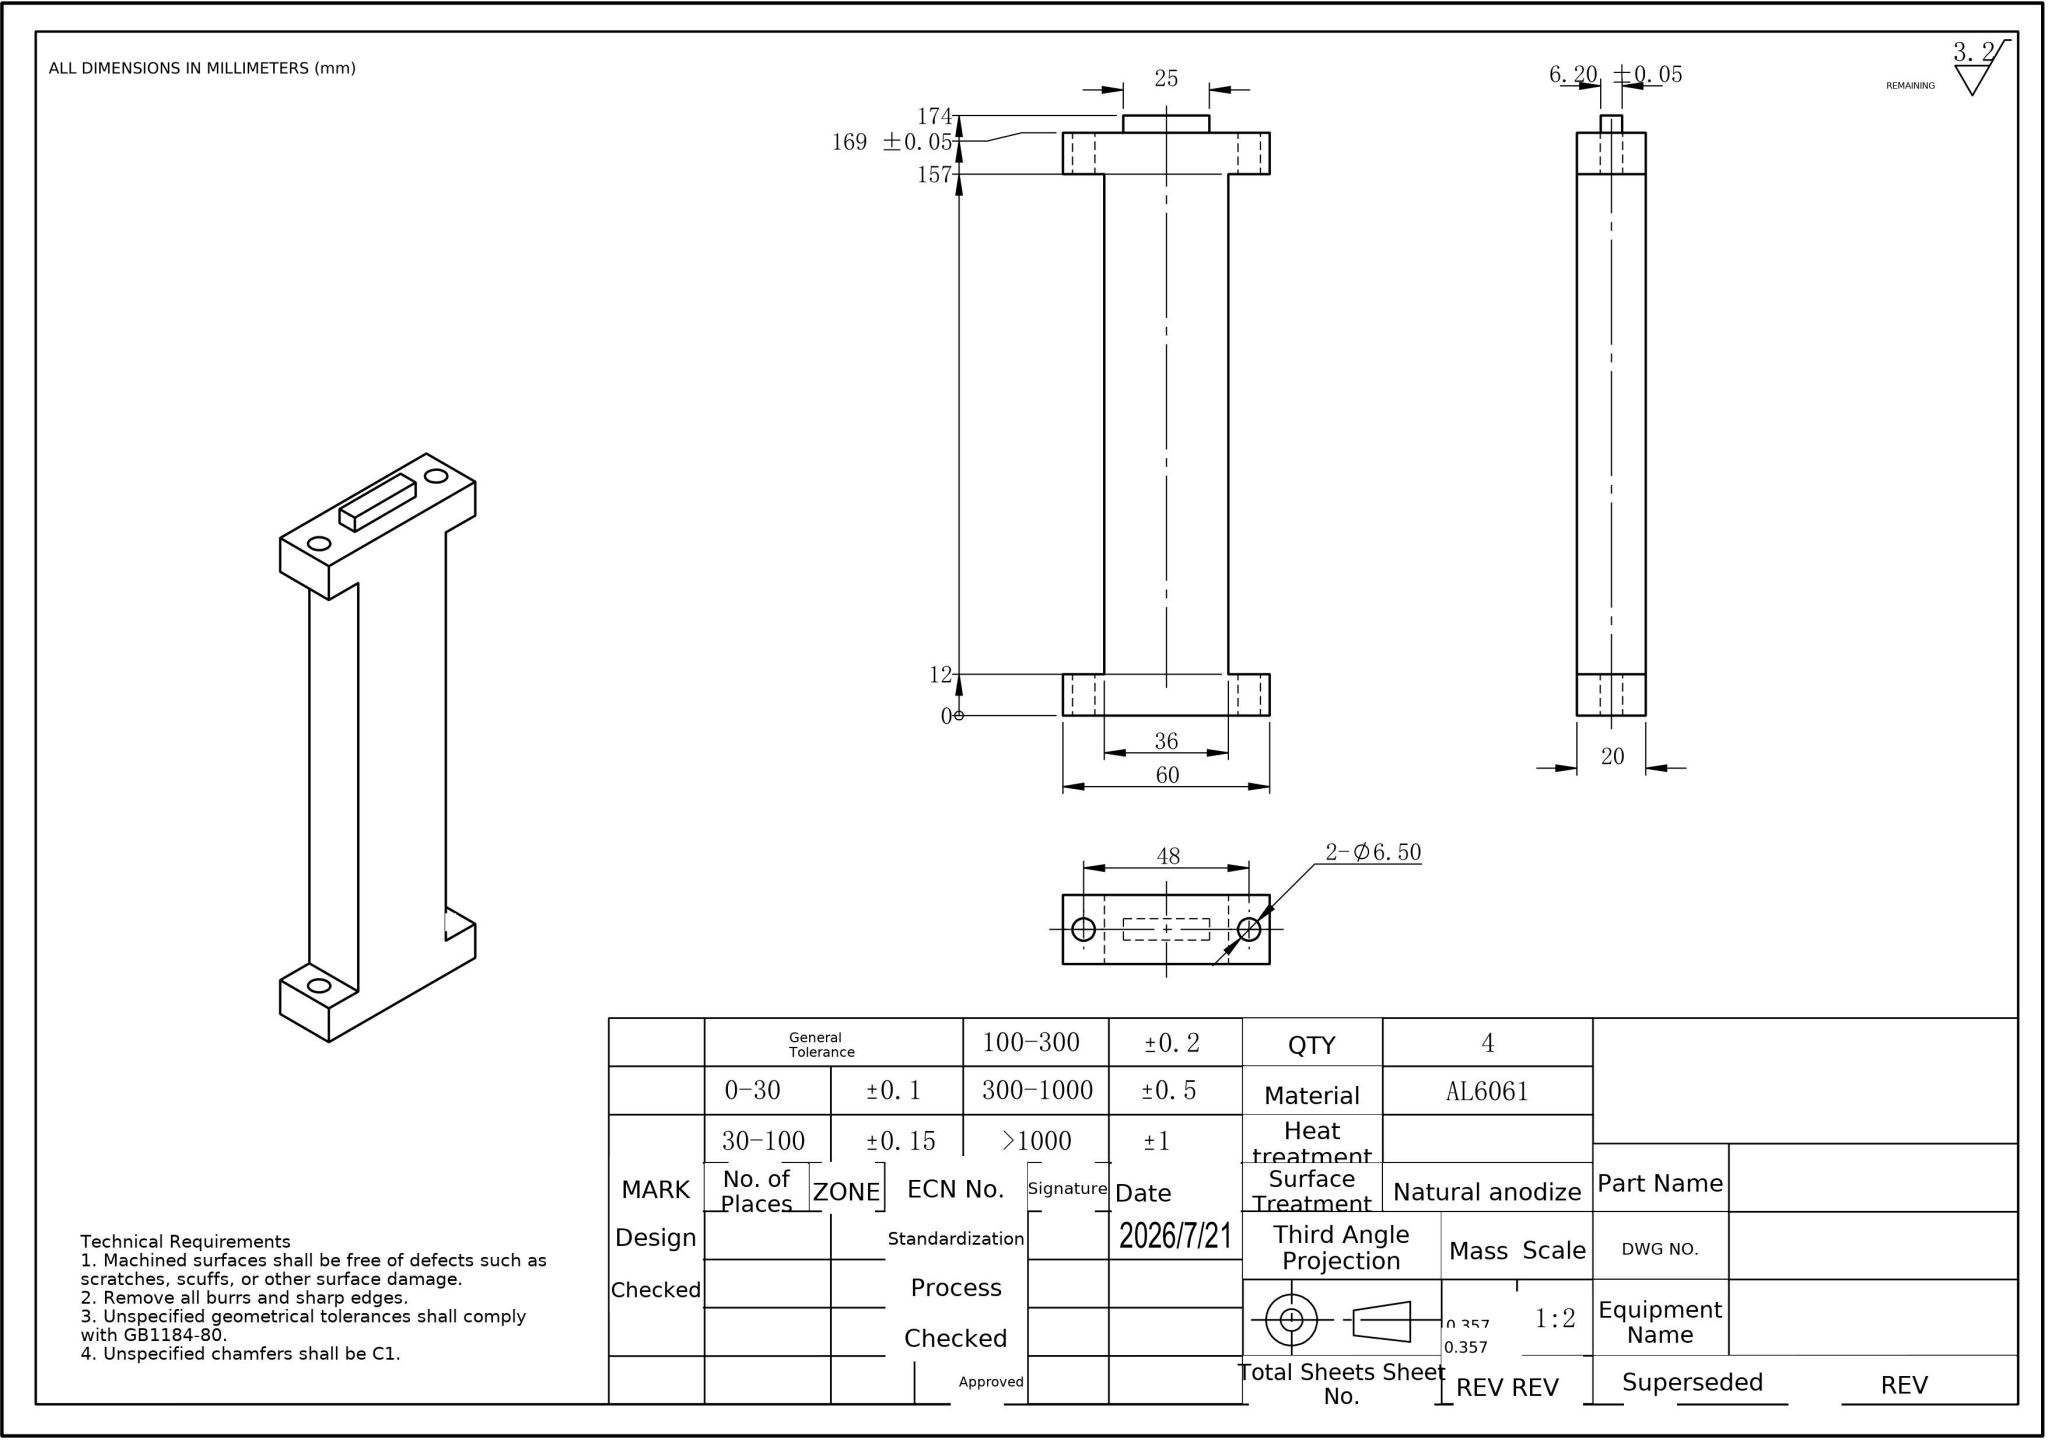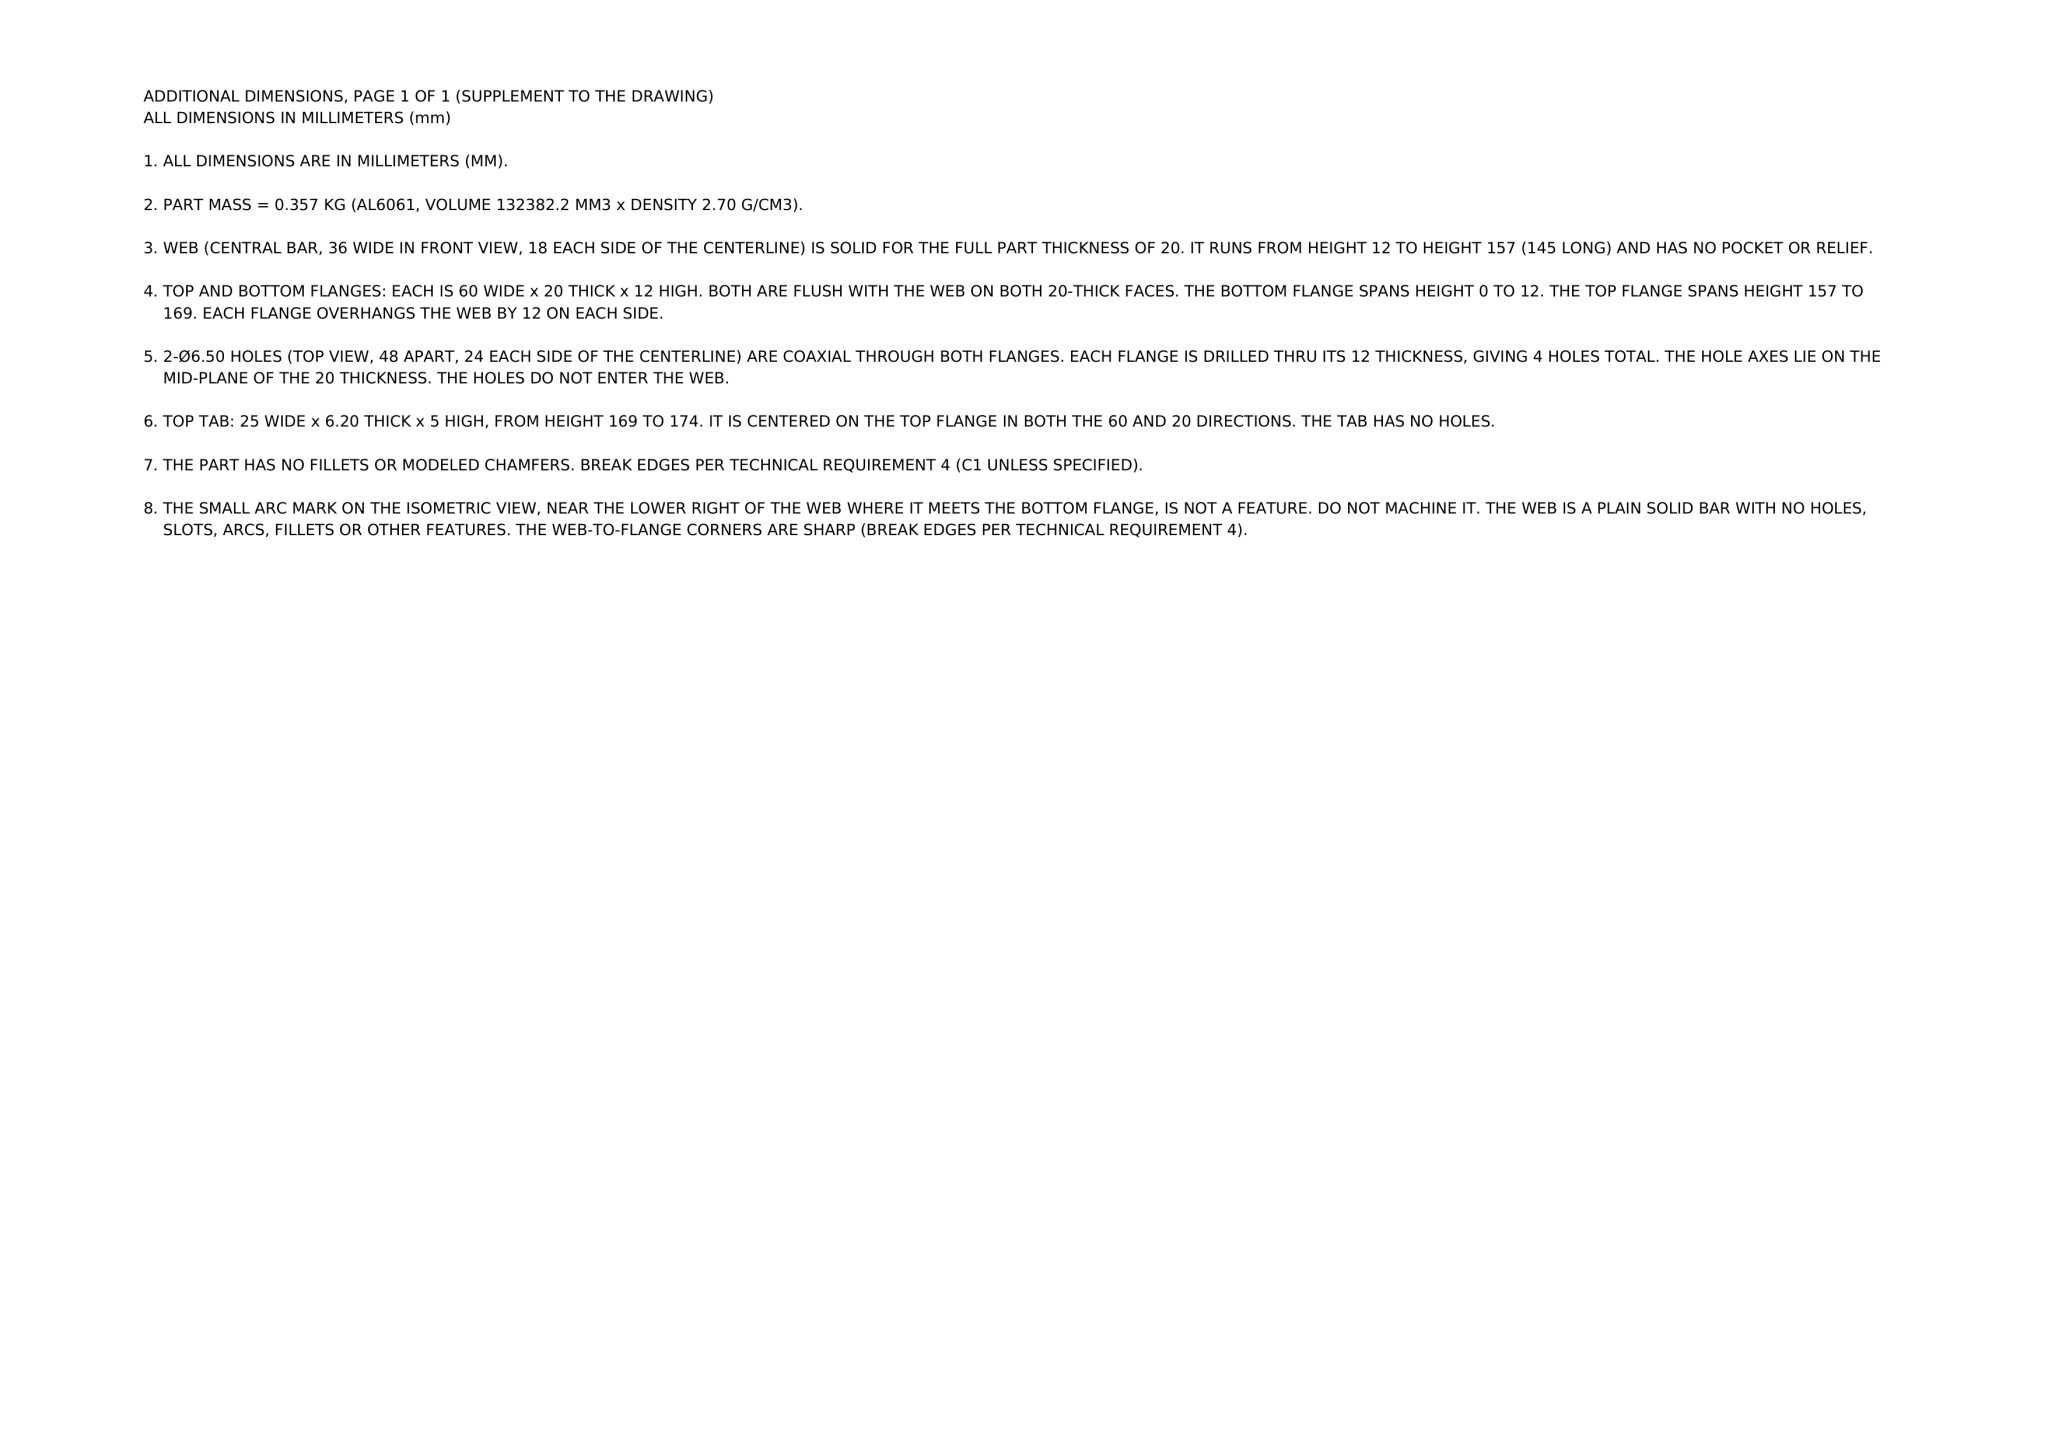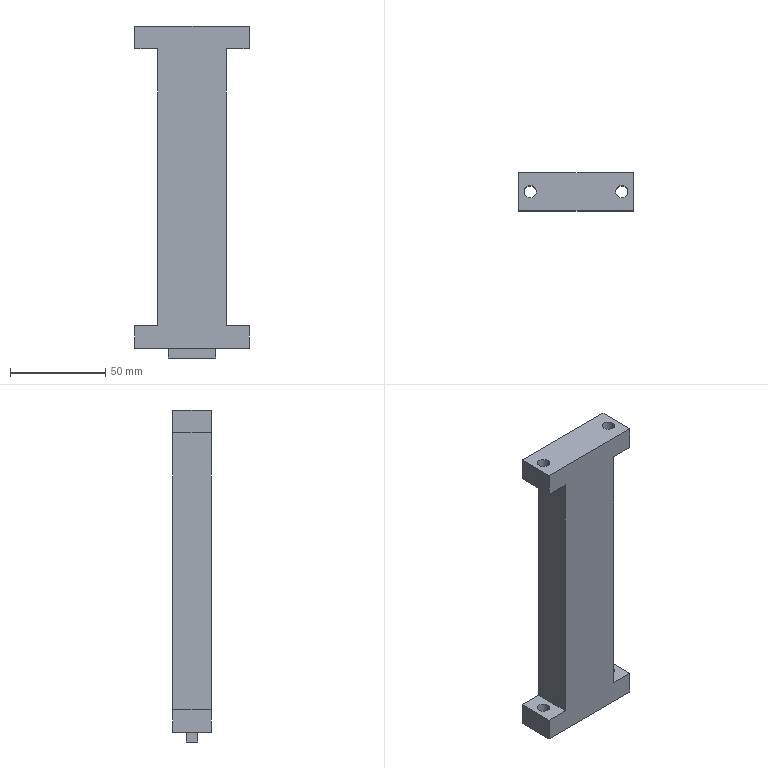Part | NX | mm | 1 solid | 27 faces | box 60 x 20 x 174 mm | volume 132382 mm3 | plane 19 | cylinder 8 | commonest cylinder face diameters 6.5 x8
STEP:
#1=COLOUR_RGB('',0.7922,0.8196,0.9333);
#2=FILL_AREA_STYLE_COLOUR('',#1);
#3=FILL_AREA_STYLE('',(#2));
#4=SURFACE_STYLE_FILL_AREA(#3);
#5=SURFACE_SIDE_STYLE('',(#4));
#6=SURFACE_STYLE_USAGE(.BOTH.,#5);
#7=PRESENTATION_STYLE_ASSIGNMENT((#6));
#8=CARTESIAN_POINT('',(27.25,-0.,-72.5));
#9=VERTEX_POINT('',#8);
#10=CARTESIAN_POINT('',(20.75,-0.,-72.5));
#11=VERTEX_POINT('',#10);
#12=CARTESIAN_POINT('',(24.,-0.,-72.5));
#13=DIRECTION('',(0.,0.,-1.));
#14=DIRECTION('',(-1.,0.,0.));
#15=AXIS2_PLACEMENT_3D('',#12,#13,#14);
#16=CIRCLE('',#15,3.25);
#17=EDGE_CURVE('',#9,#11,#16,.T.);
#18=ORIENTED_EDGE('',*,*,#17,.F.);
#19=CARTESIAN_POINT('',(27.25,-0.,-84.5));
#20=VERTEX_POINT('',#19);
#21=CARTESIAN_POINT('',(27.25,-0.,93.692));
#22=DIRECTION('',(0.,0.,-1.));
#23=VECTOR('',#22,1000.);
#24=LINE('',#21,#23);
#25=EDGE_CURVE('',#9,#20,#24,.T.);
#26=ORIENTED_EDGE('',*,*,#25,.T.);
#27=CARTESIAN_POINT('',(20.75,-0.,-84.5));
#28=VERTEX_POINT('',#27);
#29=CARTESIAN_POINT('',(24.,-0.,-84.5));
#30=DIRECTION('',(0.,0.,-1.));
#31=DIRECTION('',(1.,0.,0.));
#32=AXIS2_PLACEMENT_3D('',#29,#30,#31);
#33=CIRCLE('',#32,3.25);
#34=EDGE_CURVE('',#20,#28,#33,.T.);
#35=ORIENTED_EDGE('',*,*,#34,.T.);
#36=CARTESIAN_POINT('',(20.75,-0.,93.692));
#37=DIRECTION('',(0.,0.,-1.));
#38=VECTOR('',#37,1000.);
#39=LINE('',#36,#38);
#40=EDGE_CURVE('',#11,#28,#39,.T.);
#41=ORIENTED_EDGE('',*,*,#40,.F.);
#42=EDGE_LOOP('',(#18,#26,#35,#41));
#43=FACE_OUTER_BOUND('',#42,.T.);
#44=CARTESIAN_POINT('',(24.,-0.,93.692));
#45=DIRECTION('',(0.,0.,-1.));
#46=DIRECTION('',(-1.,0.,0.));
#47=AXIS2_PLACEMENT_3D('',#44,#45,#46);
#48=CYLINDRICAL_SURFACE('',#47,3.25);
#49=ADVANCED_FACE('',(#43),#48,.F.);
#50=CARTESIAN_POINT('',(20.75,-0.,84.5));
#51=VERTEX_POINT('',#50);
#52=CARTESIAN_POINT('',(27.25,-0.,84.5));
#53=VERTEX_POINT('',#52);
#54=CARTESIAN_POINT('',(24.,-0.,84.5));
#55=DIRECTION('',(0.,0.,1.));
#56=DIRECTION('',(-1.,0.,0.));
#57=AXIS2_PLACEMENT_3D('',#54,#55,#56);
#58=CIRCLE('',#57,3.25);
#59=EDGE_CURVE('',#51,#53,#58,.T.);
#60=ORIENTED_EDGE('',*,*,#59,.T.);
#61=CARTESIAN_POINT('',(27.25,-0.,72.5));
#62=VERTEX_POINT('',#61);
#63=CARTESIAN_POINT('',(27.25,-0.,93.692));
#64=DIRECTION('',(0.,0.,-1.));
#65=VECTOR('',#64,1000.);
#66=LINE('',#63,#65);
#67=EDGE_CURVE('',#53,#62,#66,.T.);
#68=ORIENTED_EDGE('',*,*,#67,.T.);
#69=CARTESIAN_POINT('',(20.75,-0.,72.5));
#70=VERTEX_POINT('',#69);
#71=CARTESIAN_POINT('',(24.,-0.,72.5));
#72=DIRECTION('',(-0.,0.,1.));
#73=DIRECTION('',(1.,0.,0.));
#74=AXIS2_PLACEMENT_3D('',#71,#72,#73);
#75=CIRCLE('',#74,3.25);
#76=EDGE_CURVE('',#70,#62,#75,.T.);
#77=ORIENTED_EDGE('',*,*,#76,.F.);
#78=CARTESIAN_POINT('',(20.75,-0.,93.692));
#79=DIRECTION('',(0.,0.,-1.));
#80=VECTOR('',#79,1000.);
#81=LINE('',#78,#80);
#82=EDGE_CURVE('',#51,#70,#81,.T.);
#83=ORIENTED_EDGE('',*,*,#82,.F.);
#84=EDGE_LOOP('',(#60,#68,#77,#83));
#85=FACE_OUTER_BOUND('',#84,.T.);
#86=CARTESIAN_POINT('',(24.,-0.,93.692));
#87=DIRECTION('',(0.,0.,-1.));
#88=DIRECTION('',(-1.,0.,0.));
#89=AXIS2_PLACEMENT_3D('',#86,#87,#88);
#90=CYLINDRICAL_SURFACE('',#89,3.25);
#91=ADVANCED_FACE('',(#85),#90,.F.);
#92=CARTESIAN_POINT('',(-27.25,-0.,84.5));
#93=VERTEX_POINT('',#92);
#94=CARTESIAN_POINT('',(-20.75,0.,84.5));
#95=VERTEX_POINT('',#94);
#96=CARTESIAN_POINT('',(-24.,-0.,84.5));
#97=DIRECTION('',(0.,0.,1.));
#98=DIRECTION('',(-1.,0.,0.));
#99=AXIS2_PLACEMENT_3D('',#96,#97,#98);
#100=CIRCLE('',#99,3.25);
#101=EDGE_CURVE('',#93,#95,#100,.T.);
#102=ORIENTED_EDGE('',*,*,#101,.T.);
#103=CARTESIAN_POINT('',(-20.75,0.,72.5));
#104=VERTEX_POINT('',#103);
#105=CARTESIAN_POINT('',(-20.75,0.,93.692));
#106=DIRECTION('',(0.,0.,-1.));
#107=VECTOR('',#106,1000.);
#108=LINE('',#105,#107);
#109=EDGE_CURVE('',#95,#104,#108,.T.);
#110=ORIENTED_EDGE('',*,*,#109,.T.);
#111=CARTESIAN_POINT('',(-27.25,-0.,72.5));
#112=VERTEX_POINT('',#111);
#113=CARTESIAN_POINT('',(-24.,-0.,72.5));
#114=DIRECTION('',(0.,0.,1.));
#115=DIRECTION('',(1.,0.,0.));
#116=AXIS2_PLACEMENT_3D('',#113,#114,#115);
#117=CIRCLE('',#116,3.25);
#118=EDGE_CURVE('',#112,#104,#117,.T.);
#119=ORIENTED_EDGE('',*,*,#118,.F.);
#120=CARTESIAN_POINT('',(-27.25,-0.,93.692));
#121=DIRECTION('',(0.,0.,-1.));
#122=VECTOR('',#121,1000.);
#123=LINE('',#120,#122);
#124=EDGE_CURVE('',#93,#112,#123,.T.);
#125=ORIENTED_EDGE('',*,*,#124,.F.);
#126=EDGE_LOOP('',(#102,#110,#119,#125));
#127=FACE_OUTER_BOUND('',#126,.T.);
#128=CARTESIAN_POINT('',(-24.,-0.,93.692));
#129=DIRECTION('',(0.,0.,-1.));
#130=DIRECTION('',(-1.,0.,0.));
#131=AXIS2_PLACEMENT_3D('',#128,#129,#130);
#132=CYLINDRICAL_SURFACE('',#131,3.25);
#133=ADVANCED_FACE('',(#127),#132,.F.);
#134=CARTESIAN_POINT('',(-20.75,0.,-72.5));
#135=VERTEX_POINT('',#134);
#136=CARTESIAN_POINT('',(-27.25,-0.,-72.5));
#137=VERTEX_POINT('',#136);
#138=CARTESIAN_POINT('',(-24.,-0.,-72.5));
#139=DIRECTION('',(0.,0.,-1.));
#140=DIRECTION('',(-1.,0.,0.));
#141=AXIS2_PLACEMENT_3D('',#138,#139,#140);
#142=CIRCLE('',#141,3.25);
#143=EDGE_CURVE('',#135,#137,#142,.T.);
#144=ORIENTED_EDGE('',*,*,#143,.F.);
#145=CARTESIAN_POINT('',(-20.75,0.,-84.5));
#146=VERTEX_POINT('',#145);
#147=CARTESIAN_POINT('',(-20.75,0.,93.692));
#148=DIRECTION('',(0.,0.,-1.));
#149=VECTOR('',#148,1000.);
#150=LINE('',#147,#149);
#151=EDGE_CURVE('',#135,#146,#150,.T.);
#152=ORIENTED_EDGE('',*,*,#151,.T.);
#153=CARTESIAN_POINT('',(-27.25,-0.,-84.5));
#154=VERTEX_POINT('',#153);
#155=CARTESIAN_POINT('',(-24.,-0.,-84.5));
#156=DIRECTION('',(0.,0.,-1.));
#157=DIRECTION('',(-1.,0.,0.));
#158=AXIS2_PLACEMENT_3D('',#155,#156,#157);
#159=CIRCLE('',#158,3.25);
#160=EDGE_CURVE('',#146,#154,#159,.T.);
#161=ORIENTED_EDGE('',*,*,#160,.T.);
#162=CARTESIAN_POINT('',(-27.25,-0.,93.692));
#163=DIRECTION('',(0.,0.,-1.));
#164=VECTOR('',#163,1000.);
#165=LINE('',#162,#164);
#166=EDGE_CURVE('',#137,#154,#165,.T.);
#167=ORIENTED_EDGE('',*,*,#166,.F.);
#168=EDGE_LOOP('',(#144,#152,#161,#167));
#169=FACE_OUTER_BOUND('',#168,.T.);
#170=CARTESIAN_POINT('',(-24.,-0.,93.692));
#171=DIRECTION('',(0.,0.,-1.));
#172=DIRECTION('',(-1.,0.,0.));
#173=AXIS2_PLACEMENT_3D('',#170,#171,#172);
#174=CYLINDRICAL_SURFACE('',#173,3.25);
#175=ADVANCED_FACE('',(#169),#174,.F.);
#176=CARTESIAN_POINT('',(24.,-0.,-84.5));
#177=DIRECTION('',(0.,0.,-1.));
#178=DIRECTION('',(1.,0.,0.));
#179=AXIS2_PLACEMENT_3D('',#176,#177,#178);
#180=CIRCLE('',#179,3.25);
#181=EDGE_CURVE('',#28,#20,#180,.T.);
#182=ORIENTED_EDGE('',*,*,#181,.F.);
#183=ORIENTED_EDGE('',*,*,#34,.F.);
#184=EDGE_LOOP('',(#182,#183));
#185=FACE_BOUND('',#184,.T.);
#186=CARTESIAN_POINT('',(-24.,-0.,-84.5));
#187=DIRECTION('',(0.,0.,-1.));
#188=DIRECTION('',(-1.,0.,0.));
#189=AXIS2_PLACEMENT_3D('',#186,#187,#188);
#190=CIRCLE('',#189,3.25);
#191=EDGE_CURVE('',#154,#146,#190,.T.);
#192=ORIENTED_EDGE('',*,*,#191,.F.);
#193=ORIENTED_EDGE('',*,*,#160,.F.);
#194=EDGE_LOOP('',(#192,#193));
#195=FACE_BOUND('',#194,.T.);
#196=CARTESIAN_POINT('',(30.,-10.,-84.5));
#197=VERTEX_POINT('',#196);
#198=CARTESIAN_POINT('',(-30.,-10.,-84.5));
#199=VERTEX_POINT('',#198);
#200=CARTESIAN_POINT('',(-30.,-10.,-84.5));
#201=DIRECTION('',(-1.,0.,0.));
#202=VECTOR('',#201,1000.);
#203=LINE('',#200,#202);
#204=EDGE_CURVE('',#197,#199,#203,.T.);
#205=ORIENTED_EDGE('',*,*,#204,.T.);
#206=CARTESIAN_POINT('',(-30.,10.,-84.5));
#207=VERTEX_POINT('',#206);
#208=CARTESIAN_POINT('',(-30.,10.,-84.5));
#209=DIRECTION('',(0.,-1.,0.));
#210=VECTOR('',#209,1000.);
#211=LINE('',#208,#210);
#212=EDGE_CURVE('',#207,#199,#211,.T.);
#213=ORIENTED_EDGE('',*,*,#212,.F.);
#214=CARTESIAN_POINT('',(30.,10.,-84.5));
#215=VERTEX_POINT('',#214);
#216=CARTESIAN_POINT('',(-30.,10.,-84.5));
#217=DIRECTION('',(-1.,0.,0.));
#218=VECTOR('',#217,1000.);
#219=LINE('',#216,#218);
#220=EDGE_CURVE('',#215,#207,#219,.T.);
#221=ORIENTED_EDGE('',*,*,#220,.F.);
#222=CARTESIAN_POINT('',(30.,10.,-84.5));
#223=DIRECTION('',(0.,-1.,0.));
#224=VECTOR('',#223,1000.);
#225=LINE('',#222,#224);
#226=EDGE_CURVE('',#215,#197,#225,.T.);
#227=ORIENTED_EDGE('',*,*,#226,.T.);
#228=EDGE_LOOP('',(#205,#213,#221,#227));
#229=FACE_OUTER_BOUND('',#228,.T.);
#230=CARTESIAN_POINT('',(-12.5,-3.1,-84.5));
#231=VERTEX_POINT('',#230);
#232=CARTESIAN_POINT('',(-12.5,3.1,-84.5));
#233=VERTEX_POINT('',#232);
#234=CARTESIAN_POINT('',(-12.5,-3.1,-84.5));
#235=DIRECTION('',(0.,1.,0.));
#236=VECTOR('',#235,1000.);
#237=LINE('',#234,#236);
#238=EDGE_CURVE('',#231,#233,#237,.T.);
#239=ORIENTED_EDGE('',*,*,#238,.F.);
#240=CARTESIAN_POINT('',(12.5,-3.1,-84.5));
#241=VERTEX_POINT('',#240);
#242=CARTESIAN_POINT('',(12.5,-3.1,-84.5));
#243=DIRECTION('',(-1.,0.,0.));
#244=VECTOR('',#243,1000.);
#245=LINE('',#242,#244);
#246=EDGE_CURVE('',#241,#231,#245,.T.);
#247=ORIENTED_EDGE('',*,*,#246,.F.);
#248=CARTESIAN_POINT('',(12.5,3.1,-84.5));
#249=VERTEX_POINT('',#248);
#250=CARTESIAN_POINT('',(12.5,-3.1,-84.5));
#251=DIRECTION('',(0.,-1.,0.));
#252=VECTOR('',#251,1000.);
#253=LINE('',#250,#252);
#254=EDGE_CURVE('',#249,#241,#253,.T.);
#255=ORIENTED_EDGE('',*,*,#254,.F.);
#256=CARTESIAN_POINT('',(12.5,3.1,-84.5));
#257=DIRECTION('',(1.,0.,0.));
#258=VECTOR('',#257,1000.);
#259=LINE('',#256,#258);
#260=EDGE_CURVE('',#233,#249,#259,.T.);
#261=ORIENTED_EDGE('',*,*,#260,.F.);
#262=EDGE_LOOP('',(#239,#247,#255,#261));
#263=FACE_BOUND('',#262,.T.);
#264=CARTESIAN_POINT('',(-30.,10.,-84.5));
#265=DIRECTION('',(0.,0.,1.));
#266=DIRECTION('',(1.,0.,0.));
#267=AXIS2_PLACEMENT_3D('',#264,#265,#266);
#268=PLANE('',#267);
#269=ADVANCED_FACE('',(#185,#195,#229,#263),#268,.F.);
#270=CARTESIAN_POINT('',(30.,10.,-72.5));
#271=VERTEX_POINT('',#270);
#272=CARTESIAN_POINT('',(30.,10.,84.5));
#273=DIRECTION('',(0.,0.,-1.));
#274=VECTOR('',#273,1000.);
#275=LINE('',#272,#274);
#276=EDGE_CURVE('',#271,#215,#275,.T.);
#277=ORIENTED_EDGE('',*,*,#276,.F.);
#278=CARTESIAN_POINT('',(30.,-10.,-72.5));
#279=VERTEX_POINT('',#278);
#280=CARTESIAN_POINT('',(30.,10.,-72.5));
#281=DIRECTION('',(0.,-1.,0.));
#282=VECTOR('',#281,1000.);
#283=LINE('',#280,#282);
#284=EDGE_CURVE('',#271,#279,#283,.T.);
#285=ORIENTED_EDGE('',*,*,#284,.T.);
#286=CARTESIAN_POINT('',(30.,-10.,84.5));
#287=DIRECTION('',(0.,0.,-1.));
#288=VECTOR('',#287,1000.);
#289=LINE('',#286,#288);
#290=EDGE_CURVE('',#279,#197,#289,.T.);
#291=ORIENTED_EDGE('',*,*,#290,.T.);
#292=ORIENTED_EDGE('',*,*,#226,.F.);
#293=EDGE_LOOP('',(#277,#285,#291,#292));
#294=FACE_OUTER_BOUND('',#293,.T.);
#295=CARTESIAN_POINT('',(30.,10.,84.5));
#296=DIRECTION('',(-1.,0.,0.));
#297=DIRECTION('',(0.,0.,1.));
#298=AXIS2_PLACEMENT_3D('',#295,#296,#297);
#299=PLANE('',#298);
#300=ADVANCED_FACE('',(#294),#299,.F.);
#301=CARTESIAN_POINT('',(-30.,10.,72.5));
#302=VERTEX_POINT('',#301);
#303=CARTESIAN_POINT('',(-30.,10.,84.5));
#304=VERTEX_POINT('',#303);
#305=CARTESIAN_POINT('',(-30.,10.,84.5));
#306=DIRECTION('',(0.,0.,1.));
#307=VECTOR('',#306,1000.);
#308=LINE('',#305,#307);
#309=EDGE_CURVE('',#302,#304,#308,.T.);
#310=ORIENTED_EDGE('',*,*,#309,.F.);
#311=CARTESIAN_POINT('',(-30.,-10.,72.5));
#312=VERTEX_POINT('',#311);
#313=CARTESIAN_POINT('',(-30.,10.,72.5));
#314=DIRECTION('',(0.,-1.,0.));
#315=VECTOR('',#314,1000.);
#316=LINE('',#313,#315);
#317=EDGE_CURVE('',#302,#312,#316,.T.);
#318=ORIENTED_EDGE('',*,*,#317,.T.);
#319=CARTESIAN_POINT('',(-30.,-10.,84.5));
#320=VERTEX_POINT('',#319);
#321=CARTESIAN_POINT('',(-30.,-10.,84.5));
#322=DIRECTION('',(0.,0.,1.));
#323=VECTOR('',#322,1000.);
#324=LINE('',#321,#323);
#325=EDGE_CURVE('',#312,#320,#324,.T.);
#326=ORIENTED_EDGE('',*,*,#325,.T.);
#327=CARTESIAN_POINT('',(-30.,10.,84.5));
#328=DIRECTION('',(0.,-1.,0.));
#329=VECTOR('',#328,1000.);
#330=LINE('',#327,#329);
#331=EDGE_CURVE('',#304,#320,#330,.T.);
#332=ORIENTED_EDGE('',*,*,#331,.F.);
#333=EDGE_LOOP('',(#310,#318,#326,#332));
#334=FACE_OUTER_BOUND('',#333,.T.);
#335=CARTESIAN_POINT('',(-30.,10.,84.5));
#336=DIRECTION('',(1.,0.,0.));
#337=DIRECTION('',(0.,0.,-1.));
#338=AXIS2_PLACEMENT_3D('',#335,#336,#337);
#339=PLANE('',#338);
#340=ADVANCED_FACE('',(#334),#339,.F.);
#341=CARTESIAN_POINT('',(30.,-10.,84.5));
#342=VERTEX_POINT('',#341);
#343=CARTESIAN_POINT('',(30.,-10.,72.5));
#344=VERTEX_POINT('',#343);
#345=CARTESIAN_POINT('',(30.,-10.,84.5));
#346=DIRECTION('',(0.,0.,-1.));
#347=VECTOR('',#346,1000.);
#348=LINE('',#345,#347);
#349=EDGE_CURVE('',#342,#344,#348,.T.);
#350=ORIENTED_EDGE('',*,*,#349,.T.);
#351=CARTESIAN_POINT('',(30.,10.,72.5));
#352=VERTEX_POINT('',#351);
#353=CARTESIAN_POINT('',(30.,10.,72.5));
#354=DIRECTION('',(0.,-1.,0.));
#355=VECTOR('',#354,1000.);
#356=LINE('',#353,#355);
#357=EDGE_CURVE('',#352,#344,#356,.T.);
#358=ORIENTED_EDGE('',*,*,#357,.F.);
#359=CARTESIAN_POINT('',(30.,10.,84.5));
#360=VERTEX_POINT('',#359);
#361=CARTESIAN_POINT('',(30.,10.,84.5));
#362=DIRECTION('',(0.,0.,-1.));
#363=VECTOR('',#362,1000.);
#364=LINE('',#361,#363);
#365=EDGE_CURVE('',#360,#352,#364,.T.);
#366=ORIENTED_EDGE('',*,*,#365,.F.);
#367=CARTESIAN_POINT('',(30.,10.,84.5));
#368=DIRECTION('',(0.,-1.,0.));
#369=VECTOR('',#368,1000.);
#370=LINE('',#367,#369);
#371=EDGE_CURVE('',#360,#342,#370,.T.);
#372=ORIENTED_EDGE('',*,*,#371,.T.);
#373=EDGE_LOOP('',(#350,#358,#366,#372));
#374=FACE_OUTER_BOUND('',#373,.T.);
#375=CARTESIAN_POINT('',(30.,10.,84.5));
#376=DIRECTION('',(-1.,0.,0.));
#377=DIRECTION('',(0.,0.,1.));
#378=AXIS2_PLACEMENT_3D('',#375,#376,#377);
#379=PLANE('',#378);
#380=ADVANCED_FACE('',(#374),#379,.F.);
#381=CARTESIAN_POINT('',(-30.,-10.,-72.5));
#382=VERTEX_POINT('',#381);
#383=CARTESIAN_POINT('',(-30.,-10.,84.5));
#384=DIRECTION('',(0.,0.,1.));
#385=VECTOR('',#384,1000.);
#386=LINE('',#383,#385);
#387=EDGE_CURVE('',#199,#382,#386,.T.);
#388=ORIENTED_EDGE('',*,*,#387,.T.);
#389=CARTESIAN_POINT('',(-30.,10.,-72.5));
#390=VERTEX_POINT('',#389);
#391=CARTESIAN_POINT('',(-30.,10.,-72.5));
#392=DIRECTION('',(0.,-1.,0.));
#393=VECTOR('',#392,1000.);
#394=LINE('',#391,#393);
#395=EDGE_CURVE('',#390,#382,#394,.T.);
#396=ORIENTED_EDGE('',*,*,#395,.F.);
#397=CARTESIAN_POINT('',(-30.,10.,84.5));
#398=DIRECTION('',(0.,0.,1.));
#399=VECTOR('',#398,1000.);
#400=LINE('',#397,#399);
#401=EDGE_CURVE('',#207,#390,#400,.T.);
#402=ORIENTED_EDGE('',*,*,#401,.F.);
#403=ORIENTED_EDGE('',*,*,#212,.T.);
#404=EDGE_LOOP('',(#388,#396,#402,#403));
#405=FACE_OUTER_BOUND('',#404,.T.);
#406=CARTESIAN_POINT('',(-30.,10.,84.5));
#407=DIRECTION('',(1.,0.,0.));
#408=DIRECTION('',(0.,0.,-1.));
#409=AXIS2_PLACEMENT_3D('',#406,#407,#408);
#410=PLANE('',#409);
#411=ADVANCED_FACE('',(#405),#410,.F.);
#412=ORIENTED_EDGE('',*,*,#59,.F.);
#413=CARTESIAN_POINT('',(24.,-0.,84.5));
#414=DIRECTION('',(0.,0.,1.));
#415=DIRECTION('',(-1.,0.,0.));
#416=AXIS2_PLACEMENT_3D('',#413,#414,#415);
#417=CIRCLE('',#416,3.25);
#418=EDGE_CURVE('',#53,#51,#417,.T.);
#419=ORIENTED_EDGE('',*,*,#418,.F.);
#420=EDGE_LOOP('',(#412,#419));
#421=FACE_BOUND('',#420,.T.);
#422=ORIENTED_EDGE('',*,*,#101,.F.);
#423=CARTESIAN_POINT('',(-24.,-0.,84.5));
#424=DIRECTION('',(0.,0.,1.));
#425=DIRECTION('',(-1.,0.,0.));
#426=AXIS2_PLACEMENT_3D('',#423,#424,#425);
#427=CIRCLE('',#426,3.25);
#428=EDGE_CURVE('',#95,#93,#427,.T.);
#429=ORIENTED_EDGE('',*,*,#428,.F.);
#430=EDGE_LOOP('',(#422,#429));
#431=FACE_BOUND('',#430,.T.);
#432=CARTESIAN_POINT('',(-30.,-10.,84.5));
#433=DIRECTION('',(1.,0.,0.));
#434=VECTOR('',#433,1000.);
#435=LINE('',#432,#434);
#436=EDGE_CURVE('',#320,#342,#435,.T.);
#437=ORIENTED_EDGE('',*,*,#436,.T.);
#438=ORIENTED_EDGE('',*,*,#371,.F.);
#439=CARTESIAN_POINT('',(-30.,10.,84.5));
#440=DIRECTION('',(1.,0.,0.));
#441=VECTOR('',#440,1000.);
#442=LINE('',#439,#441);
#443=EDGE_CURVE('',#304,#360,#442,.T.);
#444=ORIENTED_EDGE('',*,*,#443,.F.);
#445=ORIENTED_EDGE('',*,*,#331,.T.);
#446=EDGE_LOOP('',(#437,#438,#444,#445));
#447=FACE_OUTER_BOUND('',#446,.T.);
#448=CARTESIAN_POINT('',(-30.,10.,84.5));
#449=DIRECTION('',(0.,0.,-1.));
#450=DIRECTION('',(-1.,0.,0.));
#451=AXIS2_PLACEMENT_3D('',#448,#449,#450);
#452=PLANE('',#451);
#453=ADVANCED_FACE('',(#421,#431,#447),#452,.F.);
#454=CARTESIAN_POINT('',(18.,10.,72.5));
#455=VERTEX_POINT('',#454);
#456=CARTESIAN_POINT('',(18.,10.,-72.5));
#457=VERTEX_POINT('',#456);
#458=CARTESIAN_POINT('',(18.,10.,-72.5));
#459=DIRECTION('',(0.,0.,-1.));
#460=VECTOR('',#459,1000.);
#461=LINE('',#458,#460);
#462=EDGE_CURVE('',#455,#457,#461,.T.);
#463=ORIENTED_EDGE('',*,*,#462,.T.);
#464=CARTESIAN_POINT('',(30.,10.,-72.5));
#465=DIRECTION('',(1.,0.,0.));
#466=VECTOR('',#465,1000.);
#467=LINE('',#464,#466);
#468=EDGE_CURVE('',#457,#271,#467,.T.);
#469=ORIENTED_EDGE('',*,*,#468,.T.);
#470=ORIENTED_EDGE('',*,*,#276,.T.);
#471=ORIENTED_EDGE('',*,*,#220,.T.);
#472=ORIENTED_EDGE('',*,*,#401,.T.);
#473=CARTESIAN_POINT('',(-18.,10.,-72.5));
#474=VERTEX_POINT('',#473);
#475=CARTESIAN_POINT('',(-30.,10.,-72.5));
#476=DIRECTION('',(1.,0.,0.));
#477=VECTOR('',#476,1000.);
#478=LINE('',#475,#477);
#479=EDGE_CURVE('',#390,#474,#478,.T.);
#480=ORIENTED_EDGE('',*,*,#479,.T.);
#481=CARTESIAN_POINT('',(-18.,10.,72.5));
#482=VERTEX_POINT('',#481);
#483=CARTESIAN_POINT('',(-18.,10.,-72.5));
#484=DIRECTION('',(0.,0.,1.));
#485=VECTOR('',#484,1000.);
#486=LINE('',#483,#485);
#487=EDGE_CURVE('',#474,#482,#486,.T.);
#488=ORIENTED_EDGE('',*,*,#487,.T.);
#489=CARTESIAN_POINT('',(-30.,10.,72.5));
#490=DIRECTION('',(-1.,0.,0.));
#491=VECTOR('',#490,1000.);
#492=LINE('',#489,#491);
#493=EDGE_CURVE('',#482,#302,#492,.T.);
#494=ORIENTED_EDGE('',*,*,#493,.T.);
#495=ORIENTED_EDGE('',*,*,#309,.T.);
#496=ORIENTED_EDGE('',*,*,#443,.T.);
#497=ORIENTED_EDGE('',*,*,#365,.T.);
#498=CARTESIAN_POINT('',(30.,10.,72.5));
#499=DIRECTION('',(-1.,0.,-0.));
#500=VECTOR('',#499,1000.);
#501=LINE('',#498,#500);
#502=EDGE_CURVE('',#352,#455,#501,.T.);
#503=ORIENTED_EDGE('',*,*,#502,.T.);
#504=EDGE_LOOP('',(#463,#469,#470,#471,#472,#480,#488,#494,#495,#496,#497,#503));
#505=FACE_OUTER_BOUND('',#504,.T.);
#506=CARTESIAN_POINT('',(0.,10.,0.));
#507=DIRECTION('',(0.,-1.,0.));
#508=DIRECTION('',(0.,0.,-1.));
#509=AXIS2_PLACEMENT_3D('',#506,#507,#508);
#510=PLANE('',#509);
#511=ADVANCED_FACE('',(#505),#510,.F.);
#512=CARTESIAN_POINT('',(18.,-10.,-72.5));
#513=VERTEX_POINT('',#512);
#514=CARTESIAN_POINT('',(30.,-10.,-72.5));
#515=DIRECTION('',(1.,0.,0.));
#516=VECTOR('',#515,1000.);
#517=LINE('',#514,#516);
#518=EDGE_CURVE('',#513,#279,#517,.T.);
#519=ORIENTED_EDGE('',*,*,#518,.F.);
#520=CARTESIAN_POINT('',(18.,-10.,72.5));
#521=VERTEX_POINT('',#520);
#522=CARTESIAN_POINT('',(18.,-10.,-72.5));
#523=DIRECTION('',(0.,0.,-1.));
#524=VECTOR('',#523,1000.);
#525=LINE('',#522,#524);
#526=EDGE_CURVE('',#521,#513,#525,.T.);
#527=ORIENTED_EDGE('',*,*,#526,.F.);
#528=CARTESIAN_POINT('',(30.,-10.,72.5));
#529=DIRECTION('',(-1.,0.,-0.));
#530=VECTOR('',#529,1000.);
#531=LINE('',#528,#530);
#532=EDGE_CURVE('',#344,#521,#531,.T.);
#533=ORIENTED_EDGE('',*,*,#532,.F.);
#534=ORIENTED_EDGE('',*,*,#349,.F.);
#535=ORIENTED_EDGE('',*,*,#436,.F.);
#536=ORIENTED_EDGE('',*,*,#325,.F.);
#537=CARTESIAN_POINT('',(-18.,-10.,72.5));
#538=VERTEX_POINT('',#537);
#539=CARTESIAN_POINT('',(-30.,-10.,72.5));
#540=DIRECTION('',(-1.,0.,0.));
#541=VECTOR('',#540,1000.);
#542=LINE('',#539,#541);
#543=EDGE_CURVE('',#538,#312,#542,.T.);
#544=ORIENTED_EDGE('',*,*,#543,.F.);
#545=CARTESIAN_POINT('',(-18.,-10.,-72.5));
#546=VERTEX_POINT('',#545);
#547=CARTESIAN_POINT('',(-18.,-10.,-72.5));
#548=DIRECTION('',(0.,0.,1.));
#549=VECTOR('',#548,1000.);
#550=LINE('',#547,#549);
#551=EDGE_CURVE('',#546,#538,#550,.T.);
#552=ORIENTED_EDGE('',*,*,#551,.F.);
#553=CARTESIAN_POINT('',(-30.,-10.,-72.5));
#554=DIRECTION('',(1.,0.,0.));
#555=VECTOR('',#554,1000.);
#556=LINE('',#553,#555);
#557=EDGE_CURVE('',#382,#546,#556,.T.);
#558=ORIENTED_EDGE('',*,*,#557,.F.);
#559=ORIENTED_EDGE('',*,*,#387,.F.);
#560=ORIENTED_EDGE('',*,*,#204,.F.);
#561=ORIENTED_EDGE('',*,*,#290,.F.);
#562=EDGE_LOOP('',(#519,#527,#533,#534,#535,#536,#544,#552,#558,#559,#560,#561));
#563=FACE_OUTER_BOUND('',#562,.T.);
#564=CARTESIAN_POINT('',(0.,-10.,0.));
#565=DIRECTION('',(0.,-1.,0.));
#566=DIRECTION('',(0.,0.,-1.));
#567=AXIS2_PLACEMENT_3D('',#564,#565,#566);
#568=PLANE('',#567);
#569=ADVANCED_FACE('',(#563),#568,.T.);
#570=ORIENTED_EDGE('',*,*,#118,.T.);
#571=CARTESIAN_POINT('',(-24.,-0.,72.5));
#572=DIRECTION('',(0.,0.,1.));
#573=DIRECTION('',(1.,0.,0.));
#574=AXIS2_PLACEMENT_3D('',#571,#572,#573);
#575=CIRCLE('',#574,3.25);
#576=EDGE_CURVE('',#104,#112,#575,.T.);
#577=ORIENTED_EDGE('',*,*,#576,.T.);
#578=EDGE_LOOP('',(#570,#577));
#579=FACE_BOUND('',#578,.T.);
#580=ORIENTED_EDGE('',*,*,#543,.T.);
#581=ORIENTED_EDGE('',*,*,#317,.F.);
#582=ORIENTED_EDGE('',*,*,#493,.F.);
#583=CARTESIAN_POINT('',(-18.,10.,72.5));
#584=DIRECTION('',(0.,-1.,0.));
#585=VECTOR('',#584,1000.);
#586=LINE('',#583,#585);
#587=EDGE_CURVE('',#482,#538,#586,.T.);
#588=ORIENTED_EDGE('',*,*,#587,.T.);
#589=EDGE_LOOP('',(#580,#581,#582,#588));
#590=FACE_OUTER_BOUND('',#589,.T.);
#591=CARTESIAN_POINT('',(-30.,10.,72.5));
#592=DIRECTION('',(0.,0.,1.));
#593=DIRECTION('',(1.,0.,0.));
#594=AXIS2_PLACEMENT_3D('',#591,#592,#593);
#595=PLANE('',#594);
#596=ADVANCED_FACE('',(#579,#590),#595,.F.);
#597=ORIENTED_EDGE('',*,*,#551,.T.);
#598=ORIENTED_EDGE('',*,*,#587,.F.);
#599=ORIENTED_EDGE('',*,*,#487,.F.);
#600=CARTESIAN_POINT('',(-18.,10.,-72.5));
#601=DIRECTION('',(0.,-1.,0.));
#602=VECTOR('',#601,1000.);
#603=LINE('',#600,#602);
#604=EDGE_CURVE('',#474,#546,#603,.T.);
#605=ORIENTED_EDGE('',*,*,#604,.T.);
#606=EDGE_LOOP('',(#597,#598,#599,#605));
#607=FACE_OUTER_BOUND('',#606,.T.);
#608=CARTESIAN_POINT('',(-18.,10.,-72.5));
#609=DIRECTION('',(1.,0.,0.));
#610=DIRECTION('',(0.,0.,-1.));
#611=AXIS2_PLACEMENT_3D('',#608,#609,#610);
#612=PLANE('',#611);
#613=ADVANCED_FACE('',(#607),#612,.F.);
#614=CARTESIAN_POINT('',(-24.,-0.,-72.5));
#615=DIRECTION('',(0.,0.,-1.));
#616=DIRECTION('',(-1.,0.,0.));
#617=AXIS2_PLACEMENT_3D('',#614,#615,#616);
#618=CIRCLE('',#617,3.25);
#619=EDGE_CURVE('',#137,#135,#618,.T.);
#620=ORIENTED_EDGE('',*,*,#619,.T.);
#621=ORIENTED_EDGE('',*,*,#143,.T.);
#622=EDGE_LOOP('',(#620,#621));
#623=FACE_BOUND('',#622,.T.);
#624=ORIENTED_EDGE('',*,*,#557,.T.);
#625=ORIENTED_EDGE('',*,*,#604,.F.);
#626=ORIENTED_EDGE('',*,*,#479,.F.);
#627=ORIENTED_EDGE('',*,*,#395,.T.);
#628=EDGE_LOOP('',(#624,#625,#626,#627));
#629=FACE_OUTER_BOUND('',#628,.T.);
#630=CARTESIAN_POINT('',(-30.,10.,-72.5));
#631=DIRECTION('',(0.,0.,-1.));
#632=DIRECTION('',(-1.,0.,0.));
#633=AXIS2_PLACEMENT_3D('',#630,#631,#632);
#634=PLANE('',#633);
#635=ADVANCED_FACE('',(#623,#629),#634,.F.);
#636=CARTESIAN_POINT('',(24.,-0.,-72.5));
#637=DIRECTION('',(0.,0.,-1.));
#638=DIRECTION('',(-1.,0.,0.));
#639=AXIS2_PLACEMENT_3D('',#636,#637,#638);
#640=CIRCLE('',#639,3.25);
#641=EDGE_CURVE('',#11,#9,#640,.T.);
#642=ORIENTED_EDGE('',*,*,#641,.T.);
#643=ORIENTED_EDGE('',*,*,#17,.T.);
#644=EDGE_LOOP('',(#642,#643));
#645=FACE_BOUND('',#644,.T.);
#646=ORIENTED_EDGE('',*,*,#518,.T.);
#647=ORIENTED_EDGE('',*,*,#284,.F.);
#648=ORIENTED_EDGE('',*,*,#468,.F.);
#649=CARTESIAN_POINT('',(18.,10.,-72.5));
#650=DIRECTION('',(0.,-1.,0.));
#651=VECTOR('',#650,1000.);
#652=LINE('',#649,#651);
#653=EDGE_CURVE('',#457,#513,#652,.T.);
#654=ORIENTED_EDGE('',*,*,#653,.T.);
#655=EDGE_LOOP('',(#646,#647,#648,#654));
#656=FACE_OUTER_BOUND('',#655,.T.);
#657=CARTESIAN_POINT('',(30.,10.,-72.5));
#658=DIRECTION('',(0.,0.,-1.));
#659=DIRECTION('',(-1.,0.,-0.));
#660=AXIS2_PLACEMENT_3D('',#657,#658,#659);
#661=PLANE('',#660);
#662=ADVANCED_FACE('',(#645,#656),#661,.F.);
#663=ORIENTED_EDGE('',*,*,#526,.T.);
#664=ORIENTED_EDGE('',*,*,#653,.F.);
#665=ORIENTED_EDGE('',*,*,#462,.F.);
#666=CARTESIAN_POINT('',(18.,10.,72.5));
#667=DIRECTION('',(0.,-1.,0.));
#668=VECTOR('',#667,1000.);
#669=LINE('',#666,#668);
#670=EDGE_CURVE('',#455,#521,#669,.T.);
#671=ORIENTED_EDGE('',*,*,#670,.T.);
#672=EDGE_LOOP('',(#663,#664,#665,#671));
#673=FACE_OUTER_BOUND('',#672,.T.);
#674=CARTESIAN_POINT('',(18.,10.,-72.5));
#675=DIRECTION('',(-1.,0.,-0.));
#676=DIRECTION('',(-0.,0.,1.));
#677=AXIS2_PLACEMENT_3D('',#674,#675,#676);
#678=PLANE('',#677);
#679=ADVANCED_FACE('',(#673),#678,.F.);
#680=ORIENTED_EDGE('',*,*,#76,.T.);
#681=CARTESIAN_POINT('',(24.,-0.,72.5));
#682=DIRECTION('',(-0.,0.,1.));
#683=DIRECTION('',(1.,0.,0.));
#684=AXIS2_PLACEMENT_3D('',#681,#682,#683);
#685=CIRCLE('',#684,3.25);
#686=EDGE_CURVE('',#62,#70,#685,.T.);
#687=ORIENTED_EDGE('',*,*,#686,.T.);
#688=EDGE_LOOP('',(#680,#687));
#689=FACE_BOUND('',#688,.T.);
#690=ORIENTED_EDGE('',*,*,#532,.T.);
#691=ORIENTED_EDGE('',*,*,#670,.F.);
#692=ORIENTED_EDGE('',*,*,#502,.F.);
#693=ORIENTED_EDGE('',*,*,#357,.T.);
#694=EDGE_LOOP('',(#690,#691,#692,#693));
#695=FACE_OUTER_BOUND('',#694,.T.);
#696=CARTESIAN_POINT('',(30.,10.,72.5));
#697=DIRECTION('',(-0.,0.,1.));
#698=DIRECTION('',(1.,0.,0.));
#699=AXIS2_PLACEMENT_3D('',#696,#697,#698);
#700=PLANE('',#699);
#701=ADVANCED_FACE('',(#689,#695),#700,.F.);
#702=ORIENTED_EDGE('',*,*,#238,.T.);
#703=CARTESIAN_POINT('',(-12.5,3.1,-89.5));
#704=VERTEX_POINT('',#703);
#705=CARTESIAN_POINT('',(-12.5,3.1,-89.5));
#706=DIRECTION('',(0.,0.,1.));
#707=VECTOR('',#706,1000.);
#708=LINE('',#705,#707);
#709=EDGE_CURVE('',#704,#233,#708,.T.);
#710=ORIENTED_EDGE('',*,*,#709,.F.);
#711=CARTESIAN_POINT('',(-12.5,-3.1,-89.5));
#712=VERTEX_POINT('',#711);
#713=CARTESIAN_POINT('',(-12.5,-3.1,-89.5));
#714=DIRECTION('',(0.,1.,0.));
#715=VECTOR('',#714,1000.);
#716=LINE('',#713,#715);
#717=EDGE_CURVE('',#712,#704,#716,.T.);
#718=ORIENTED_EDGE('',*,*,#717,.F.);
#719=CARTESIAN_POINT('',(-12.5,-3.1,-89.5));
#720=DIRECTION('',(0.,0.,1.));
#721=VECTOR('',#720,1000.);
#722=LINE('',#719,#721);
#723=EDGE_CURVE('',#712,#231,#722,.T.);
#724=ORIENTED_EDGE('',*,*,#723,.T.);
#725=EDGE_LOOP('',(#702,#710,#718,#724));
#726=FACE_OUTER_BOUND('',#725,.T.);
#727=CARTESIAN_POINT('',(-12.5,-3.1,-89.5));
#728=DIRECTION('',(1.,0.,0.));
#729=DIRECTION('',(0.,0.,-1.));
#730=AXIS2_PLACEMENT_3D('',#727,#728,#729);
#731=PLANE('',#730);
#732=ADVANCED_FACE('',(#726),#731,.F.);
#733=ORIENTED_EDGE('',*,*,#260,.T.);
#734=CARTESIAN_POINT('',(12.5,3.1,-89.5));
#735=VERTEX_POINT('',#734);
#736=CARTESIAN_POINT('',(12.5,3.1,-89.5));
#737=DIRECTION('',(0.,0.,1.));
#738=VECTOR('',#737,1000.);
#739=LINE('',#736,#738);
#740=EDGE_CURVE('',#735,#249,#739,.T.);
#741=ORIENTED_EDGE('',*,*,#740,.F.);
#742=CARTESIAN_POINT('',(12.5,3.1,-89.5));
#743=DIRECTION('',(1.,0.,0.));
#744=VECTOR('',#743,1000.);
#745=LINE('',#742,#744);
#746=EDGE_CURVE('',#704,#735,#745,.T.);
#747=ORIENTED_EDGE('',*,*,#746,.F.);
#748=ORIENTED_EDGE('',*,*,#709,.T.);
#749=EDGE_LOOP('',(#733,#741,#747,#748));
#750=FACE_OUTER_BOUND('',#749,.T.);
#751=CARTESIAN_POINT('',(12.5,3.1,-89.5));
#752=DIRECTION('',(0.,-1.,0.));
#753=DIRECTION('',(0.,0.,-1.));
#754=AXIS2_PLACEMENT_3D('',#751,#752,#753);
#755=PLANE('',#754);
#756=ADVANCED_FACE('',(#750),#755,.F.);
#757=ORIENTED_EDGE('',*,*,#254,.T.);
#758=CARTESIAN_POINT('',(12.5,-3.1,-89.5));
#759=VERTEX_POINT('',#758);
#760=CARTESIAN_POINT('',(12.5,-3.1,-89.5));
#761=DIRECTION('',(0.,0.,1.));
#762=VECTOR('',#761,1000.);
#763=LINE('',#760,#762);
#764=EDGE_CURVE('',#759,#241,#763,.T.);
#765=ORIENTED_EDGE('',*,*,#764,.F.);
#766=CARTESIAN_POINT('',(12.5,-3.1,-89.5));
#767=DIRECTION('',(0.,-1.,0.));
#768=VECTOR('',#767,1000.);
#769=LINE('',#766,#768);
#770=EDGE_CURVE('',#735,#759,#769,.T.);
#771=ORIENTED_EDGE('',*,*,#770,.F.);
#772=ORIENTED_EDGE('',*,*,#740,.T.);
#773=EDGE_LOOP('',(#757,#765,#771,#772));
#774=FACE_OUTER_BOUND('',#773,.T.);
#775=CARTESIAN_POINT('',(12.5,-3.1,-89.5));
#776=DIRECTION('',(-1.,0.,0.));
#777=DIRECTION('',(0.,0.,1.));
#778=AXIS2_PLACEMENT_3D('',#775,#776,#777);
#779=PLANE('',#778);
#780=ADVANCED_FACE('',(#774),#779,.F.);
#781=ORIENTED_EDGE('',*,*,#246,.T.);
#782=ORIENTED_EDGE('',*,*,#723,.F.);
#783=CARTESIAN_POINT('',(12.5,-3.1,-89.5));
#784=DIRECTION('',(-1.,0.,0.));
#785=VECTOR('',#784,1000.);
#786=LINE('',#783,#785);
#787=EDGE_CURVE('',#759,#712,#786,.T.);
#788=ORIENTED_EDGE('',*,*,#787,.F.);
#789=ORIENTED_EDGE('',*,*,#764,.T.);
#790=EDGE_LOOP('',(#781,#782,#788,#789));
#791=FACE_OUTER_BOUND('',#790,.T.);
#792=CARTESIAN_POINT('',(12.5,-3.1,-89.5));
#793=DIRECTION('',(0.,1.,0.));
#794=DIRECTION('',(0.,0.,1.));
#795=AXIS2_PLACEMENT_3D('',#792,#793,#794);
#796=PLANE('',#795);
#797=ADVANCED_FACE('',(#791),#796,.F.);
#798=ORIENTED_EDGE('',*,*,#717,.T.);
#799=ORIENTED_EDGE('',*,*,#746,.T.);
#800=ORIENTED_EDGE('',*,*,#770,.T.);
#801=ORIENTED_EDGE('',*,*,#787,.T.);
#802=EDGE_LOOP('',(#798,#799,#800,#801));
#803=FACE_OUTER_BOUND('',#802,.T.);
#804=CARTESIAN_POINT('',(0.,0.,-89.5));
#805=DIRECTION('',(0.,0.,1.));
#806=DIRECTION('',(1.,0.,0.));
#807=AXIS2_PLACEMENT_3D('',#804,#805,#806);
#808=PLANE('',#807);
#809=ADVANCED_FACE('',(#803),#808,.F.);
#810=ORIENTED_EDGE('',*,*,#151,.F.);
#811=ORIENTED_EDGE('',*,*,#619,.F.);
#812=ORIENTED_EDGE('',*,*,#166,.T.);
#813=ORIENTED_EDGE('',*,*,#191,.T.);
#814=EDGE_LOOP('',(#810,#811,#812,#813));
#815=FACE_OUTER_BOUND('',#814,.T.);
#816=CARTESIAN_POINT('',(-24.,-0.,93.692));
#817=DIRECTION('',(0.,0.,-1.));
#818=DIRECTION('',(-1.,0.,0.));
#819=AXIS2_PLACEMENT_3D('',#816,#817,#818);
#820=CYLINDRICAL_SURFACE('',#819,3.25);
#821=ADVANCED_FACE('',(#815),#820,.F.);
#822=ORIENTED_EDGE('',*,*,#109,.F.);
#823=ORIENTED_EDGE('',*,*,#428,.T.);
#824=ORIENTED_EDGE('',*,*,#124,.T.);
#825=ORIENTED_EDGE('',*,*,#576,.F.);
#826=EDGE_LOOP('',(#822,#823,#824,#825));
#827=FACE_OUTER_BOUND('',#826,.T.);
#828=CARTESIAN_POINT('',(-24.,-0.,93.692));
#829=DIRECTION('',(0.,0.,-1.));
#830=DIRECTION('',(-1.,0.,0.));
#831=AXIS2_PLACEMENT_3D('',#828,#829,#830);
#832=CYLINDRICAL_SURFACE('',#831,3.25);
#833=ADVANCED_FACE('',(#827),#832,.F.);
#834=ORIENTED_EDGE('',*,*,#67,.F.);
#835=ORIENTED_EDGE('',*,*,#418,.T.);
#836=ORIENTED_EDGE('',*,*,#82,.T.);
#837=ORIENTED_EDGE('',*,*,#686,.F.);
#838=EDGE_LOOP('',(#834,#835,#836,#837));
#839=FACE_OUTER_BOUND('',#838,.T.);
#840=CARTESIAN_POINT('',(24.,-0.,93.692));
#841=DIRECTION('',(0.,0.,-1.));
#842=DIRECTION('',(-1.,0.,0.));
#843=AXIS2_PLACEMENT_3D('',#840,#841,#842);
#844=CYLINDRICAL_SURFACE('',#843,3.25);
#845=ADVANCED_FACE('',(#839),#844,.F.);
#846=ORIENTED_EDGE('',*,*,#25,.F.);
#847=ORIENTED_EDGE('',*,*,#641,.F.);
#848=ORIENTED_EDGE('',*,*,#40,.T.);
#849=ORIENTED_EDGE('',*,*,#181,.T.);
#850=EDGE_LOOP('',(#846,#847,#848,#849));
#851=FACE_OUTER_BOUND('',#850,.T.);
#852=CARTESIAN_POINT('',(24.,-0.,93.692));
#853=DIRECTION('',(0.,0.,-1.));
#854=DIRECTION('',(-1.,0.,0.));
#855=AXIS2_PLACEMENT_3D('',#852,#853,#854);
#856=CYLINDRICAL_SURFACE('',#855,3.25);
#857=ADVANCED_FACE('',(#851),#856,.F.);
#858=CLOSED_SHELL('',(#49,#91,#133,#175,#269,#300,#340,#380,#411,#453,#511,#569,#596,#613,#635,#662,#679,#701,#732,#756,#780,#797,#809,#821,#833,#845,#857));
#859=MANIFOLD_SOLID_BREP('',#858);
#860=STYLED_ITEM('',(#7),#859);
#861=(LENGTH_UNIT()NAMED_UNIT(*)SI_UNIT(.MILLI.,.METRE.));
#862=UNCERTAINTY_MEASURE_WITH_UNIT(LENGTH_MEASURE(0.00001),#861,'','');
#863=(NAMED_UNIT(*)PLANE_ANGLE_UNIT()SI_UNIT($,.RADIAN.));
#864=(NAMED_UNIT(*)SI_UNIT($,.STERADIAN.)SOLID_ANGLE_UNIT());
#865=(GEOMETRIC_REPRESENTATION_CONTEXT(3)GLOBAL_UNCERTAINTY_ASSIGNED_CONTEXT((#862))GLOBAL_UNIT_ASSIGNED_CONTEXT((#861,#863,#864))REPRESENTATION_CONTEXT('',''));
#866=MECHANICAL_DESIGN_GEOMETRIC_PRESENTATION_REPRESENTATION('',(#860),#865);
#867=CARTESIAN_POINT('',(0.,0.,0.));
#868=DIRECTION('',(0.,0.,1.));
#869=DIRECTION('',(1.,0.,0.));
#870=AXIS2_PLACEMENT_3D('',#867,#868,#869);
#871=(LENGTH_UNIT()NAMED_UNIT(*)SI_UNIT(.MILLI.,.METRE.));
#872=UNCERTAINTY_MEASURE_WITH_UNIT(LENGTH_MEASURE(0.00001),#871,'','');
#873=(NAMED_UNIT(*)PLANE_ANGLE_UNIT()SI_UNIT($,.RADIAN.));
#874=(NAMED_UNIT(*)SI_UNIT($,.STERADIAN.)SOLID_ANGLE_UNIT());
#875=(GEOMETRIC_REPRESENTATION_CONTEXT(3)GLOBAL_UNCERTAINTY_ASSIGNED_CONTEXT((#872))GLOBAL_UNIT_ASSIGNED_CONTEXT((#871,#873,#874))REPRESENTATION_CONTEXT('',''));
#876=ADVANCED_BREP_SHAPE_REPRESENTATION('',(#859,#870),#875);
#877=PRESENTATION_LAYER_ASSIGNMENT('','',(#860));